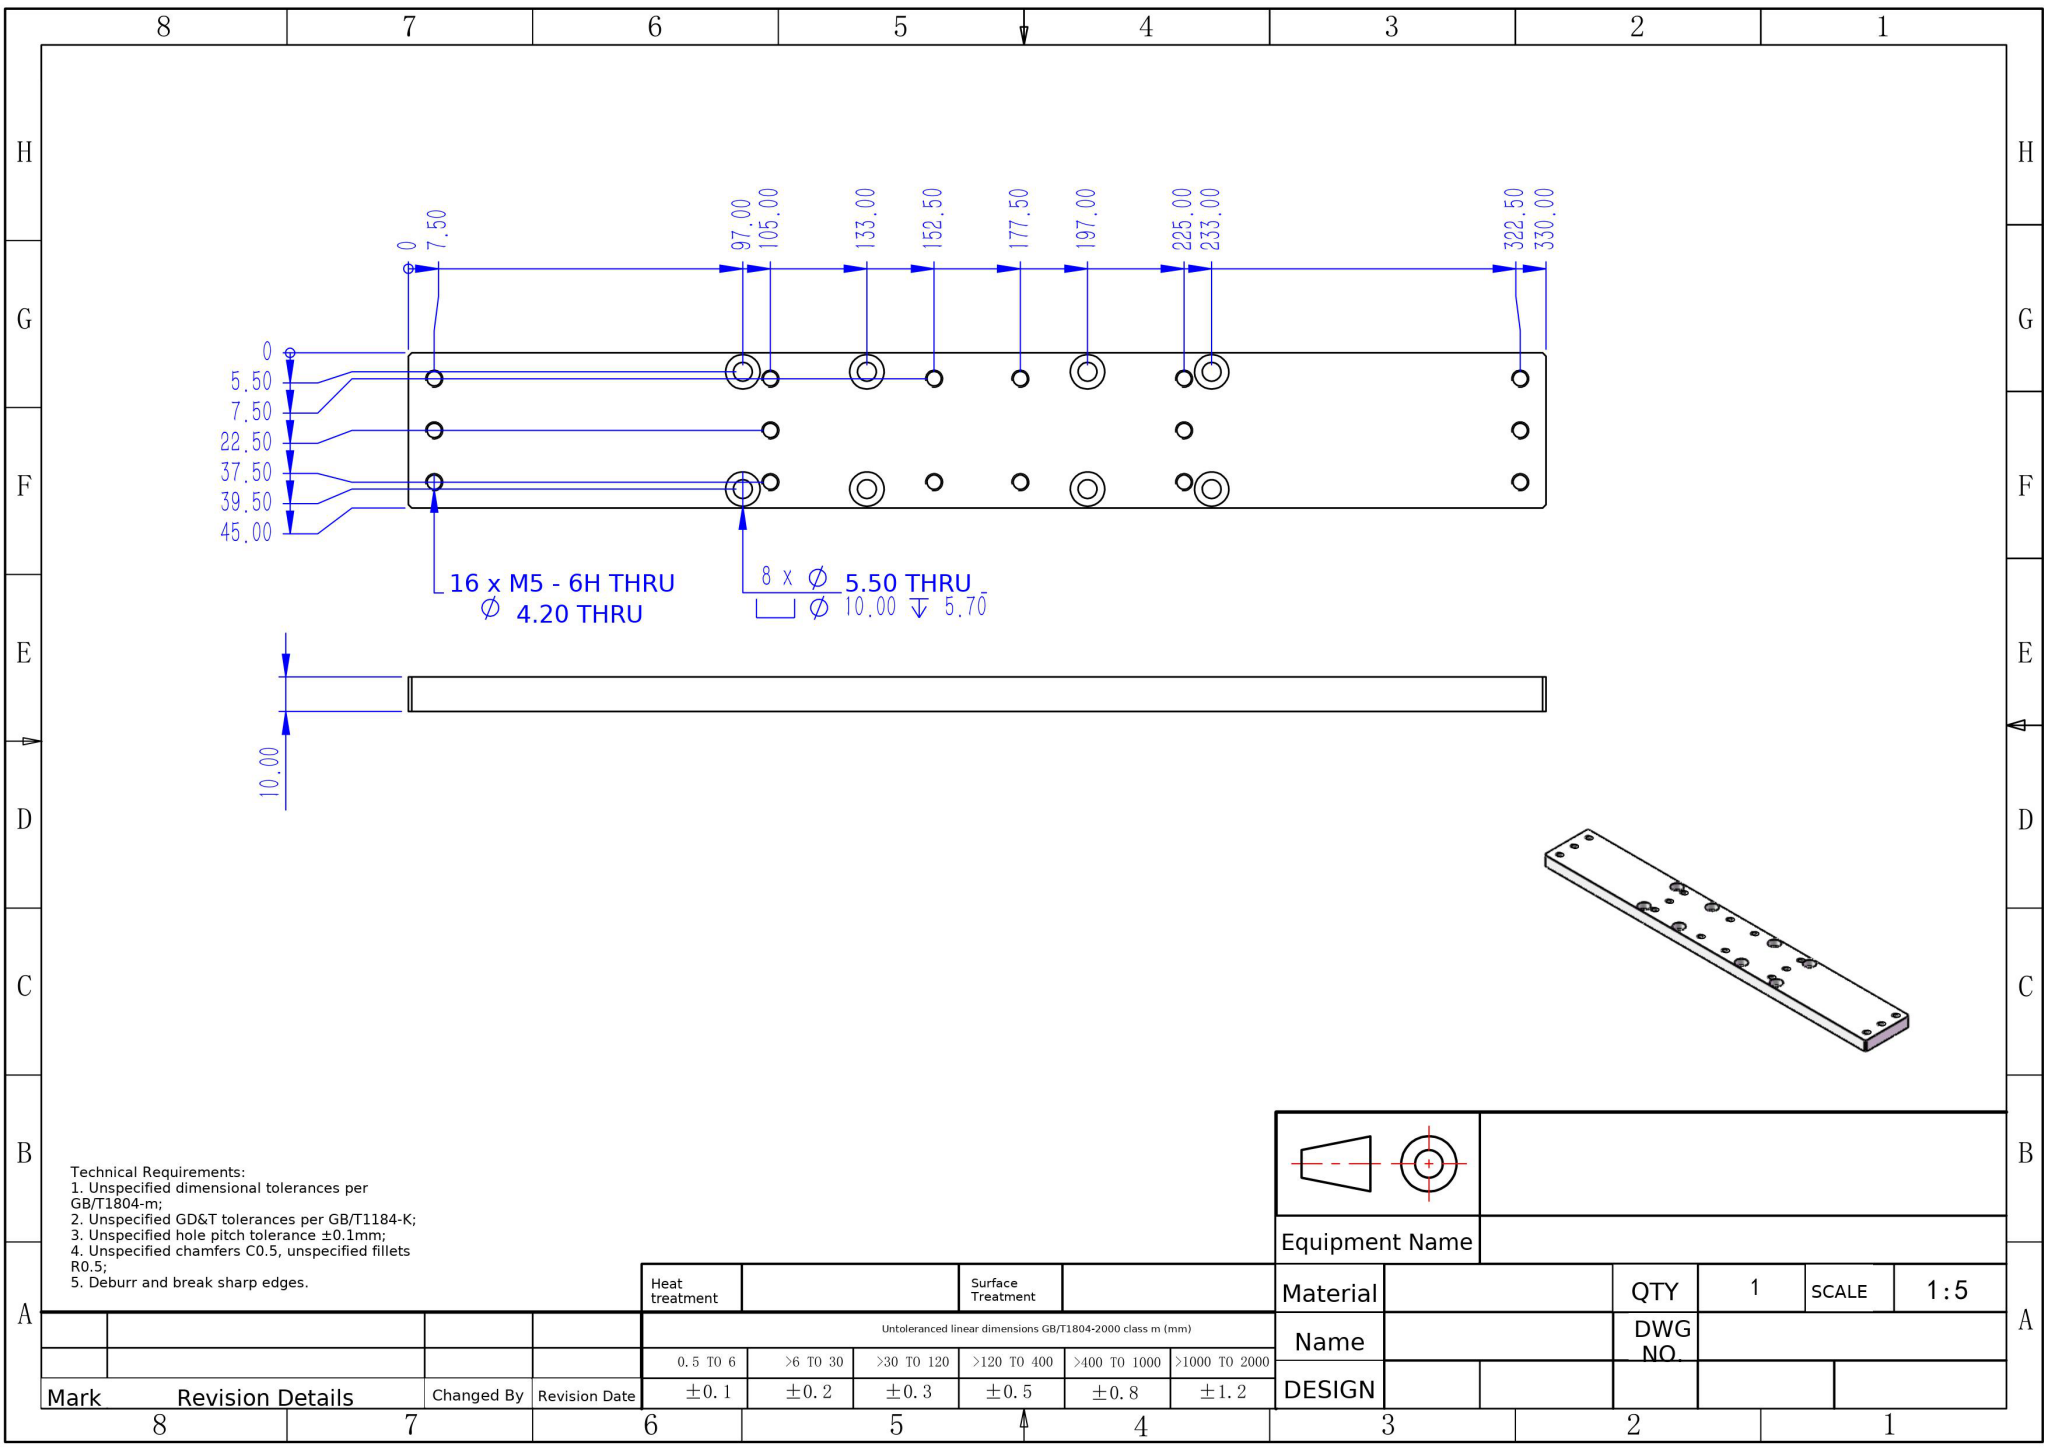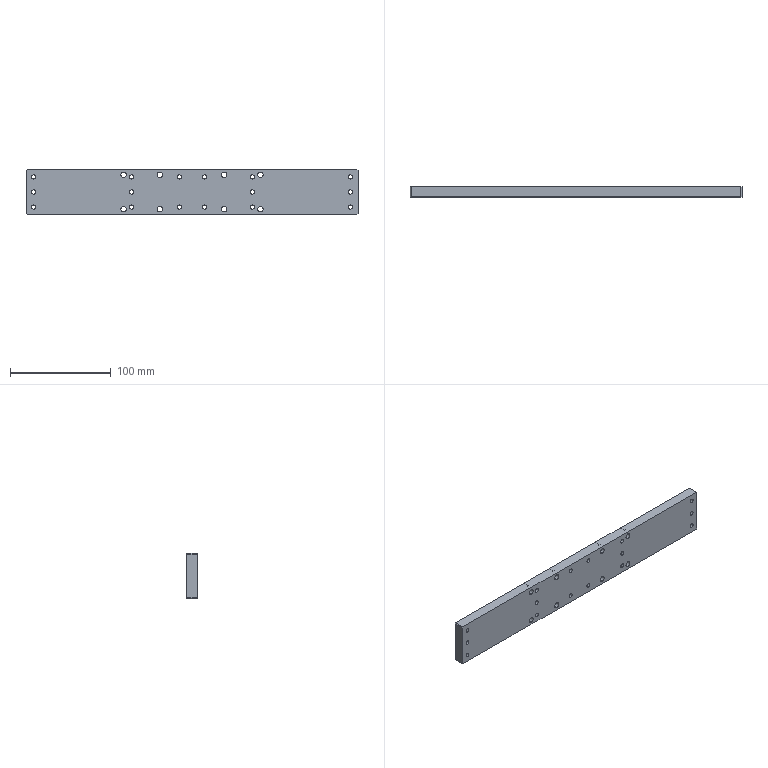Part | NX | mm | 1 solid | 82 faces | box 330 x 10 x 45 mm | volume 141865 mm3 | cylinder 64 | plane 18 | commonest cylinder face diameters 4.2 x32 10 x16 5.5 x16